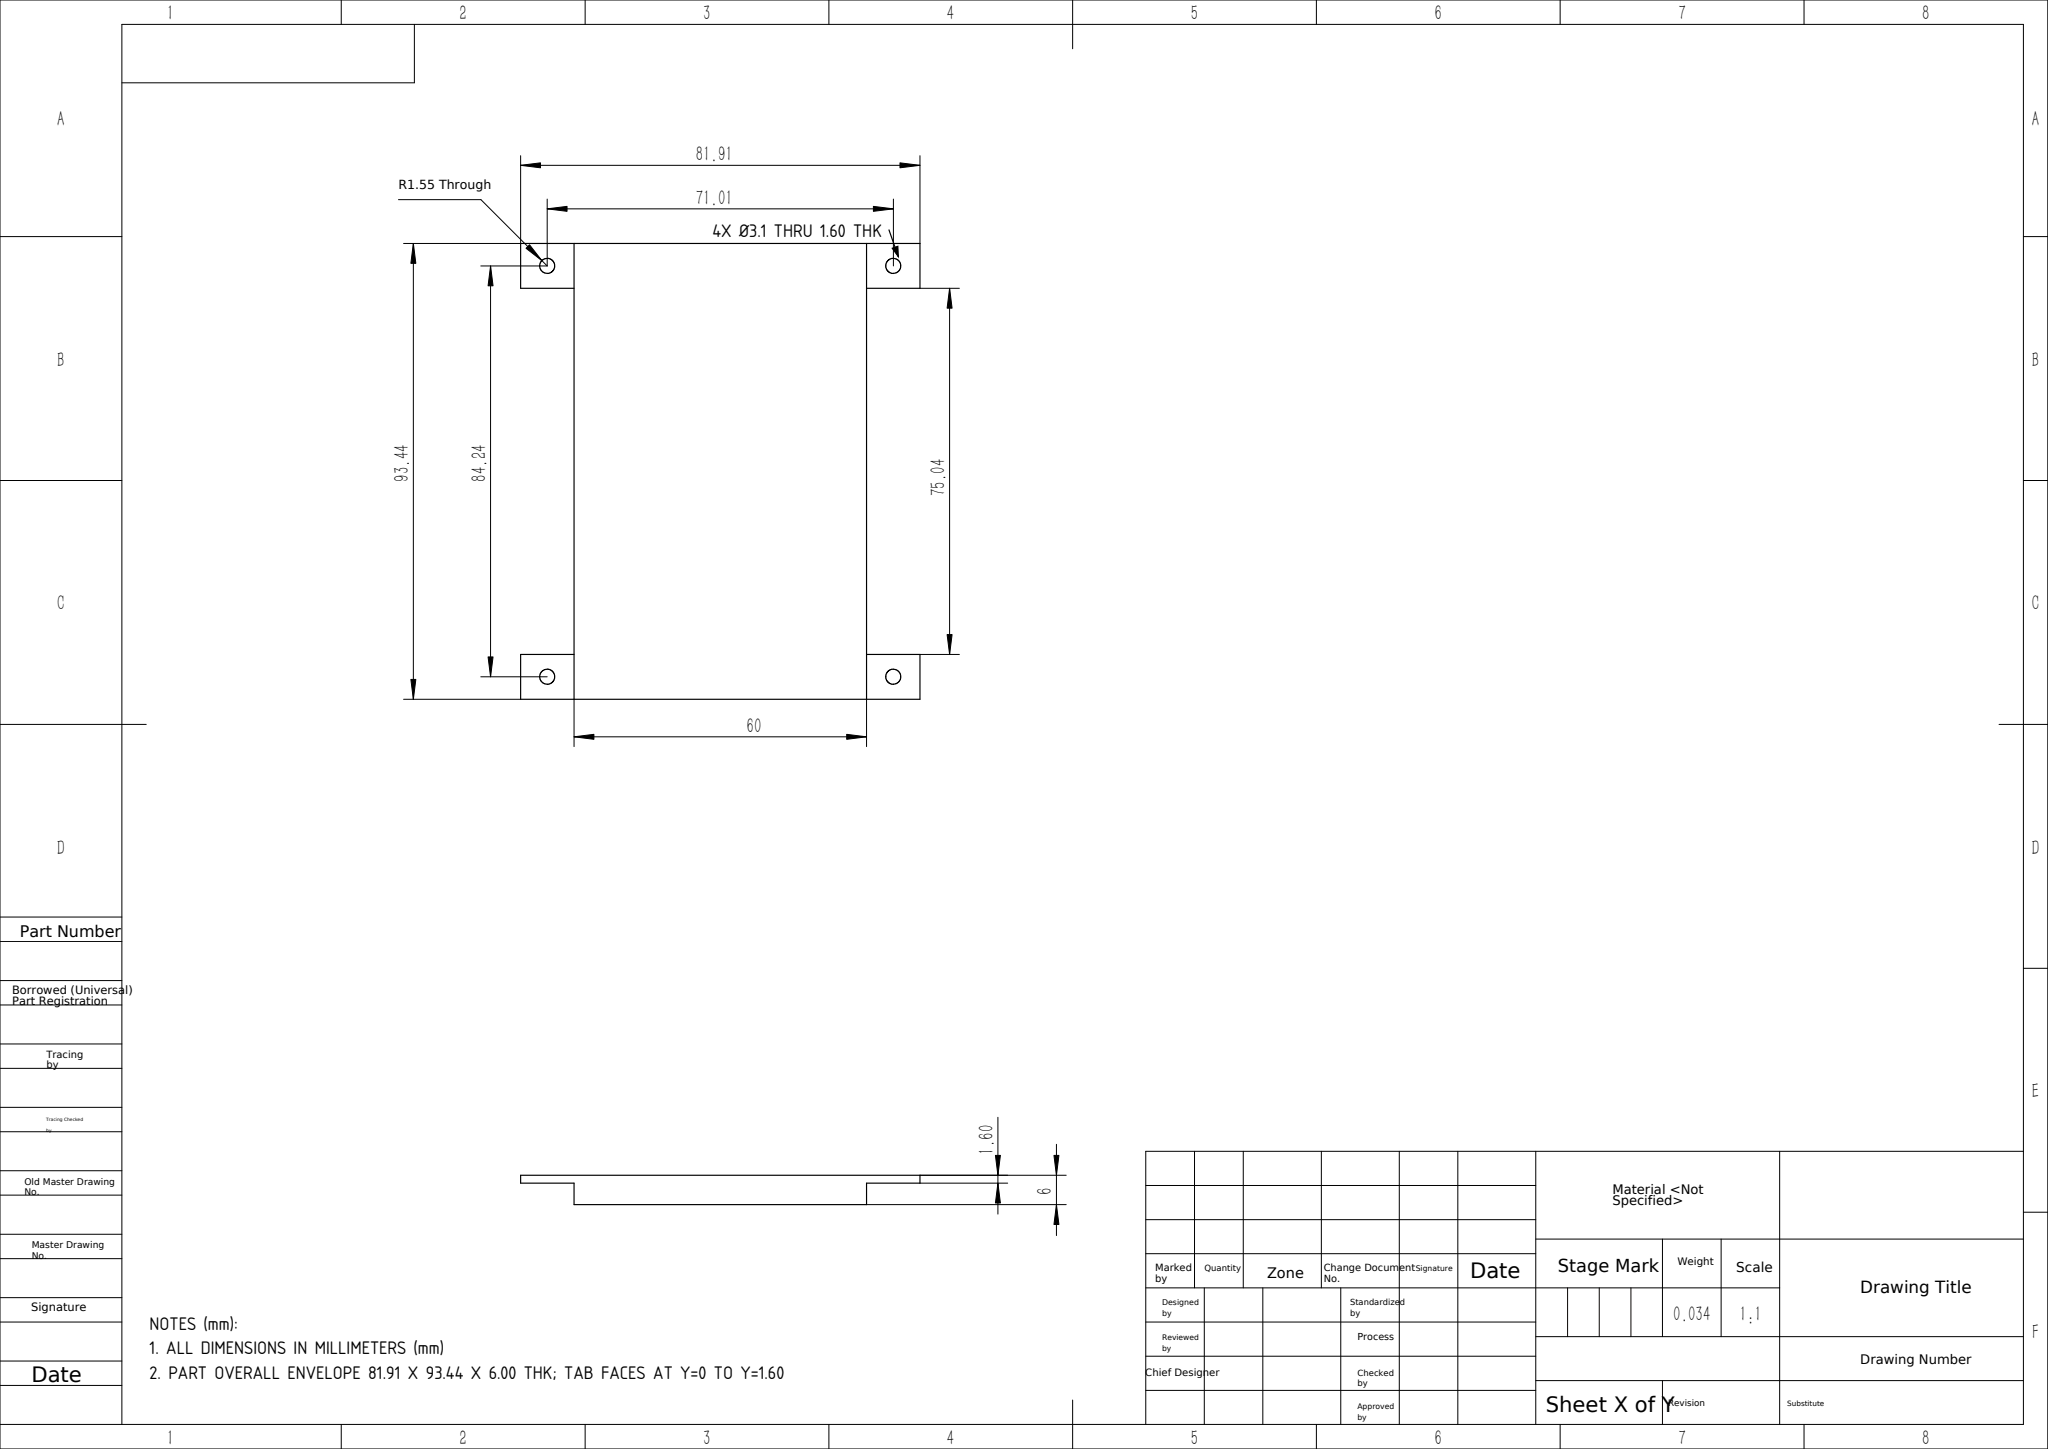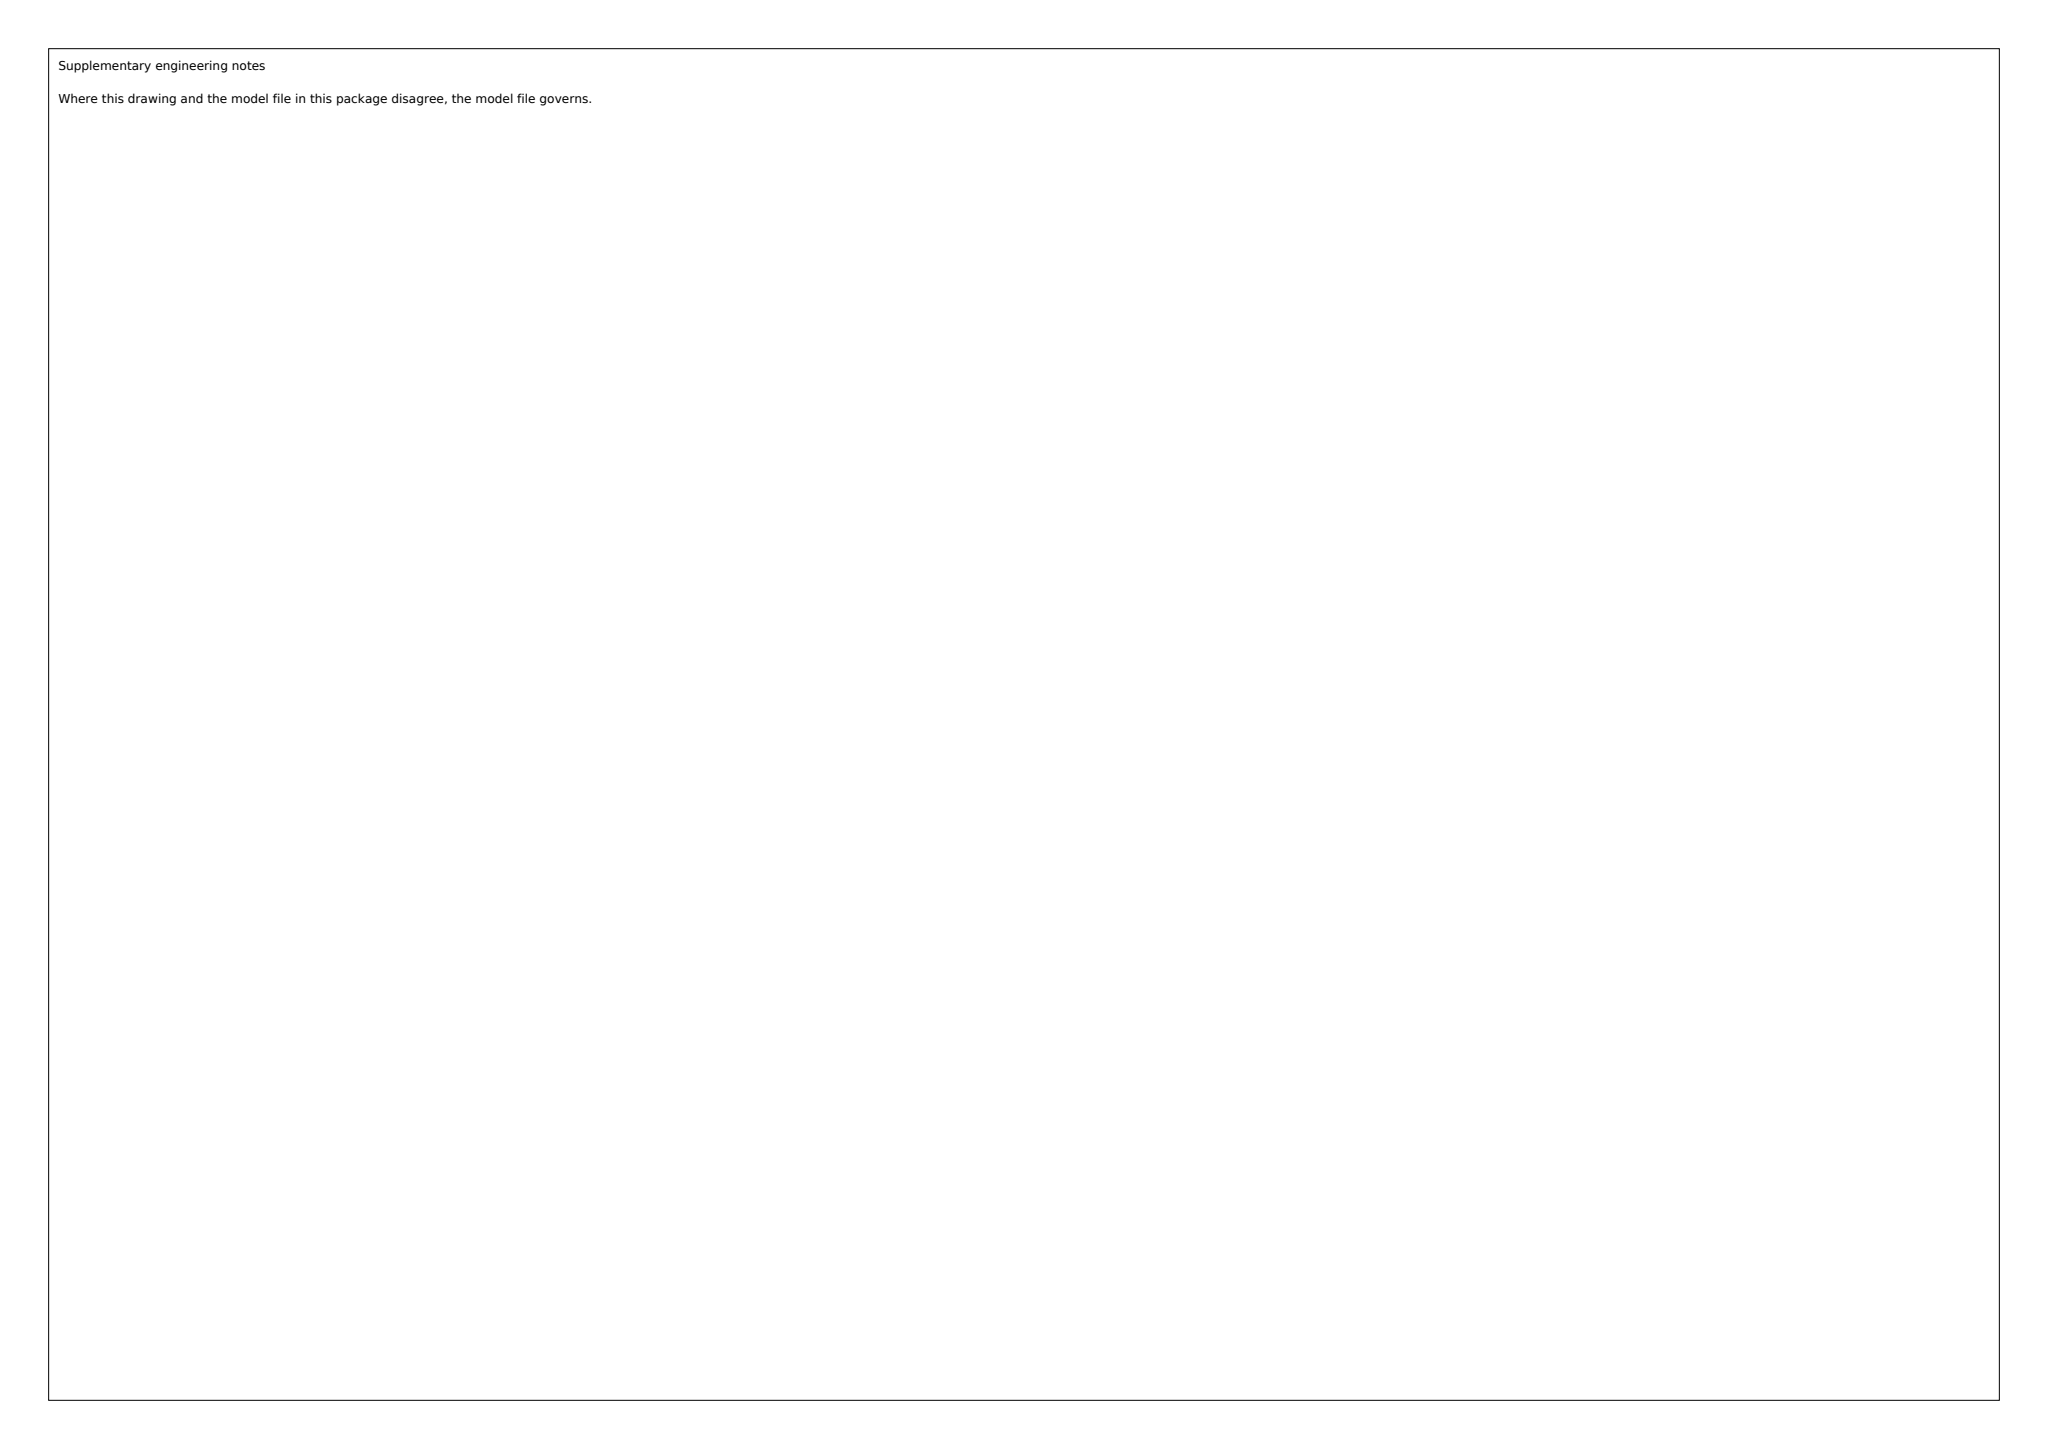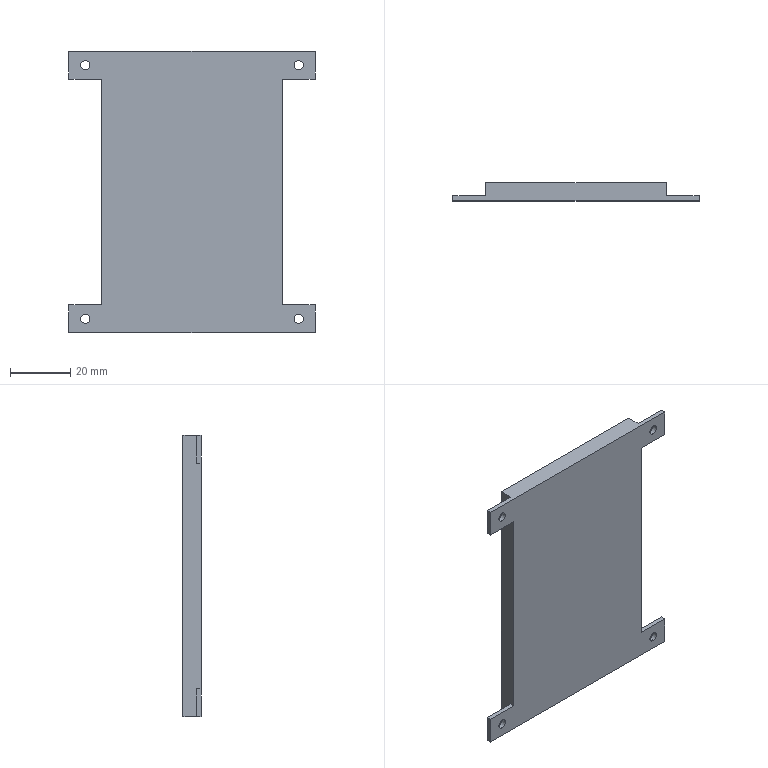Part | SolidWorks | mm | 1 solid | 26 faces | box 81.91 x 6 x 93.44 mm | volume 34235 mm3 | plane 18 | cylinder 8 | commonest cylinder face diameters 3.1 x8
Drawing notes:
ALL DIMENSIONS IN MILLIMETERS (mm) | from the solid: STEP bbox_xyz [81.91, 6.0, 93.44] given in mm
4X Ø3.1 THRU 1.60 THK MOUNTING TABS; HOLE CENTERS AT X=5.45 AND X=76.46 FROM LEFT EDGE, Z=4.60 AND Z=88.84 FROM BOTTOM EDGE | from the solid: cylinders dia 3.1, axis y, length 1.6 at (5.45,4.6), (5.45,88.84), (76.46,4.6), (76.46,88.84)
PART OVERALL ENVELOPE 81.91 X 93.44 X 6.00 THK; TAB FACES AT Y=0 TO Y=1.60 | from the solid: bbox_xyz [81.91, 6.0, 93.44]; y planes at 0.0, 1.6, 6.0
STEP:
#1=CARTESIAN_POINT('',(-35.505,0.,-43.67));
#2=VERTEX_POINT('',#1);
#3=CARTESIAN_POINT('',(-35.505,1.6,-43.67));
#4=VERTEX_POINT('',#3);
#5=CARTESIAN_POINT('',(-35.505,0.,-43.67));
#6=DIRECTION('',(0.,1.,0.));
#7=VECTOR('',#6,1000.);
#8=LINE('',#5,#7);
#9=EDGE_CURVE('',#2,#4,#8,.T.);
#10=ORIENTED_EDGE('',*,*,#9,.F.);
#11=CARTESIAN_POINT('',(-35.505,0.,-40.57));
#12=VERTEX_POINT('',#11);
#13=CARTESIAN_POINT('',(-35.505,0.,-42.12));
#14=DIRECTION('',(0.,-1.,0.));
#15=DIRECTION('',(0.,0.,1.));
#16=AXIS2_PLACEMENT_3D('',#13,#14,#15);
#17=CIRCLE('',#16,1.55);
#18=EDGE_CURVE('',#2,#12,#17,.T.);
#19=ORIENTED_EDGE('',*,*,#18,.T.);
#20=CARTESIAN_POINT('',(-35.505,1.6,-40.57));
#21=VERTEX_POINT('',#20);
#22=CARTESIAN_POINT('',(-35.505,0.,-40.57));
#23=DIRECTION('',(0.,1.,0.));
#24=VECTOR('',#23,1000.);
#25=LINE('',#22,#24);
#26=EDGE_CURVE('',#12,#21,#25,.T.);
#27=ORIENTED_EDGE('',*,*,#26,.T.);
#28=CARTESIAN_POINT('',(-35.505,1.6,-42.12));
#29=DIRECTION('',(0.,-1.,0.));
#30=DIRECTION('',(0.,0.,1.));
#31=AXIS2_PLACEMENT_3D('',#28,#29,#30);
#32=CIRCLE('',#31,1.55);
#33=EDGE_CURVE('',#4,#21,#32,.T.);
#34=ORIENTED_EDGE('',*,*,#33,.F.);
#35=EDGE_LOOP('',(#10,#19,#27,#34));
#36=FACE_OUTER_BOUND('',#35,.T.);
#37=CARTESIAN_POINT('',(-35.505,0.,-42.12));
#38=DIRECTION('',(0.,1.,0.));
#39=DIRECTION('',(0.,0.,1.));
#40=AXIS2_PLACEMENT_3D('',#37,#38,#39);
#41=CYLINDRICAL_SURFACE('',#40,1.55);
#42=ADVANCED_FACE('',(#36),#41,.F.);
#43=CARTESIAN_POINT('',(-35.505,0.,40.57));
#44=VERTEX_POINT('',#43);
#45=CARTESIAN_POINT('',(-35.505,1.6,40.57));
#46=VERTEX_POINT('',#45);
#47=CARTESIAN_POINT('',(-35.505,0.,40.57));
#48=DIRECTION('',(0.,1.,0.));
#49=VECTOR('',#48,1000.);
#50=LINE('',#47,#49);
#51=EDGE_CURVE('',#44,#46,#50,.T.);
#52=ORIENTED_EDGE('',*,*,#51,.F.);
#53=CARTESIAN_POINT('',(-35.505,0.,43.67));
#54=VERTEX_POINT('',#53);
#55=CARTESIAN_POINT('',(-35.505,0.,42.12));
#56=DIRECTION('',(0.,1.,0.));
#57=DIRECTION('',(0.,0.,-1.));
#58=AXIS2_PLACEMENT_3D('',#55,#56,#57);
#59=CIRCLE('',#58,1.55);
#60=EDGE_CURVE('',#54,#44,#59,.T.);
#61=ORIENTED_EDGE('',*,*,#60,.F.);
#62=CARTESIAN_POINT('',(-35.505,1.6,43.67));
#63=VERTEX_POINT('',#62);
#64=CARTESIAN_POINT('',(-35.505,0.,43.67));
#65=DIRECTION('',(0.,1.,0.));
#66=VECTOR('',#65,1000.);
#67=LINE('',#64,#66);
#68=EDGE_CURVE('',#54,#63,#67,.T.);
#69=ORIENTED_EDGE('',*,*,#68,.T.);
#70=CARTESIAN_POINT('',(-35.505,1.6,42.12));
#71=DIRECTION('',(0.,1.,0.));
#72=DIRECTION('',(0.,0.,-1.));
#73=AXIS2_PLACEMENT_3D('',#70,#71,#72);
#74=CIRCLE('',#73,1.55);
#75=EDGE_CURVE('',#63,#46,#74,.T.);
#76=ORIENTED_EDGE('',*,*,#75,.T.);
#77=EDGE_LOOP('',(#52,#61,#69,#76));
#78=FACE_OUTER_BOUND('',#77,.T.);
#79=CARTESIAN_POINT('',(-35.505,0.,42.12));
#80=DIRECTION('',(0.,1.,0.));
#81=DIRECTION('',(0.,0.,1.));
#82=AXIS2_PLACEMENT_3D('',#79,#80,#81);
#83=CYLINDRICAL_SURFACE('',#82,1.55);
#84=ADVANCED_FACE('',(#78),#83,.F.);
#85=CARTESIAN_POINT('',(35.505,0.,40.57));
#86=VERTEX_POINT('',#85);
#87=CARTESIAN_POINT('',(35.505,1.6,40.57));
#88=VERTEX_POINT('',#87);
#89=CARTESIAN_POINT('',(35.505,0.,40.57));
#90=DIRECTION('',(0.,1.,0.));
#91=VECTOR('',#90,1000.);
#92=LINE('',#89,#91);
#93=EDGE_CURVE('',#86,#88,#92,.T.);
#94=ORIENTED_EDGE('',*,*,#93,.F.);
#95=CARTESIAN_POINT('',(35.505,0.,43.67));
#96=VERTEX_POINT('',#95);
#97=CARTESIAN_POINT('',(35.505,0.,42.12));
#98=DIRECTION('',(0.,-1.,0.));
#99=DIRECTION('',(0.,0.,-1.));
#100=AXIS2_PLACEMENT_3D('',#97,#98,#99);
#101=CIRCLE('',#100,1.55);
#102=EDGE_CURVE('',#86,#96,#101,.T.);
#103=ORIENTED_EDGE('',*,*,#102,.T.);
#104=CARTESIAN_POINT('',(35.505,1.6,43.67));
#105=VERTEX_POINT('',#104);
#106=CARTESIAN_POINT('',(35.505,0.,43.67));
#107=DIRECTION('',(0.,1.,0.));
#108=VECTOR('',#107,1000.);
#109=LINE('',#106,#108);
#110=EDGE_CURVE('',#96,#105,#109,.T.);
#111=ORIENTED_EDGE('',*,*,#110,.T.);
#112=CARTESIAN_POINT('',(35.505,1.6,42.12));
#113=DIRECTION('',(0.,-1.,0.));
#114=DIRECTION('',(0.,0.,-1.));
#115=AXIS2_PLACEMENT_3D('',#112,#113,#114);
#116=CIRCLE('',#115,1.55);
#117=EDGE_CURVE('',#88,#105,#116,.T.);
#118=ORIENTED_EDGE('',*,*,#117,.F.);
#119=EDGE_LOOP('',(#94,#103,#111,#118));
#120=FACE_OUTER_BOUND('',#119,.T.);
#121=CARTESIAN_POINT('',(35.505,0.,42.12));
#122=DIRECTION('',(0.,1.,0.));
#123=DIRECTION('',(0.,0.,1.));
#124=AXIS2_PLACEMENT_3D('',#121,#122,#123);
#125=CYLINDRICAL_SURFACE('',#124,1.55);
#126=ADVANCED_FACE('',(#120),#125,.F.);
#127=CARTESIAN_POINT('',(35.505,0.,-43.67));
#128=VERTEX_POINT('',#127);
#129=CARTESIAN_POINT('',(35.505,1.6,-43.67));
#130=VERTEX_POINT('',#129);
#131=CARTESIAN_POINT('',(35.505,0.,-43.67));
#132=DIRECTION('',(0.,1.,0.));
#133=VECTOR('',#132,1000.);
#134=LINE('',#131,#133);
#135=EDGE_CURVE('',#128,#130,#134,.T.);
#136=ORIENTED_EDGE('',*,*,#135,.F.);
#137=CARTESIAN_POINT('',(35.505,0.,-40.57));
#138=VERTEX_POINT('',#137);
#139=CARTESIAN_POINT('',(35.505,0.,-42.12));
#140=DIRECTION('',(0.,1.,0.));
#141=DIRECTION('',(0.,0.,1.));
#142=AXIS2_PLACEMENT_3D('',#139,#140,#141);
#143=CIRCLE('',#142,1.55);
#144=EDGE_CURVE('',#138,#128,#143,.T.);
#145=ORIENTED_EDGE('',*,*,#144,.F.);
#146=CARTESIAN_POINT('',(35.505,1.6,-40.57));
#147=VERTEX_POINT('',#146);
#148=CARTESIAN_POINT('',(35.505,0.,-40.57));
#149=DIRECTION('',(0.,1.,0.));
#150=VECTOR('',#149,1000.);
#151=LINE('',#148,#150);
#152=EDGE_CURVE('',#138,#147,#151,.T.);
#153=ORIENTED_EDGE('',*,*,#152,.T.);
#154=CARTESIAN_POINT('',(35.505,1.6,-42.12));
#155=DIRECTION('',(0.,1.,0.));
#156=DIRECTION('',(0.,0.,1.));
#157=AXIS2_PLACEMENT_3D('',#154,#155,#156);
#158=CIRCLE('',#157,1.55);
#159=EDGE_CURVE('',#147,#130,#158,.T.);
#160=ORIENTED_EDGE('',*,*,#159,.T.);
#161=EDGE_LOOP('',(#136,#145,#153,#160));
#162=FACE_OUTER_BOUND('',#161,.T.);
#163=CARTESIAN_POINT('',(35.505,0.,-42.12));
#164=DIRECTION('',(0.,1.,0.));
#165=DIRECTION('',(0.,0.,1.));
#166=AXIS2_PLACEMENT_3D('',#163,#164,#165);
#167=CYLINDRICAL_SURFACE('',#166,1.55);
#168=ADVANCED_FACE('',(#162),#167,.F.);
#169=ORIENTED_EDGE('',*,*,#75,.F.);
#170=CARTESIAN_POINT('',(-35.505,1.6,42.12));
#171=DIRECTION('',(0.,1.,0.));
#172=DIRECTION('',(0.,0.,-1.));
#173=AXIS2_PLACEMENT_3D('',#170,#171,#172);
#174=CIRCLE('',#173,1.55);
#175=EDGE_CURVE('',#46,#63,#174,.T.);
#176=ORIENTED_EDGE('',*,*,#175,.F.);
#177=EDGE_LOOP('',(#169,#176));
#178=FACE_BOUND('',#177,.T.);
#179=CARTESIAN_POINT('',(-40.955,1.6,37.52));
#180=VERTEX_POINT('',#179);
#181=CARTESIAN_POINT('',(-30.,1.6,37.52));
#182=VERTEX_POINT('',#181);
#183=CARTESIAN_POINT('',(0.,1.6,37.52));
#184=DIRECTION('',(1.,0.,0.));
#185=VECTOR('',#184,1000.);
#186=LINE('',#183,#185);
#187=EDGE_CURVE('',#180,#182,#186,.T.);
#188=ORIENTED_EDGE('',*,*,#187,.F.);
#189=CARTESIAN_POINT('',(-40.955,1.6,46.72));
#190=VERTEX_POINT('',#189);
#191=CARTESIAN_POINT('',(-40.955,1.6,0.));
#192=DIRECTION('',(0.,0.,-1.));
#193=VECTOR('',#192,1000.);
#194=LINE('',#191,#193);
#195=EDGE_CURVE('',#190,#180,#194,.T.);
#196=ORIENTED_EDGE('',*,*,#195,.F.);
#197=CARTESIAN_POINT('',(-30.,1.6,46.72));
#198=VERTEX_POINT('',#197);
#199=CARTESIAN_POINT('',(0.,1.6,46.72));
#200=DIRECTION('',(-1.,0.,0.));
#201=VECTOR('',#200,1000.);
#202=LINE('',#199,#201);
#203=EDGE_CURVE('',#198,#190,#202,.T.);
#204=ORIENTED_EDGE('',*,*,#203,.F.);
#205=CARTESIAN_POINT('',(-30.,1.6,0.));
#206=DIRECTION('',(0.,0.,1.));
#207=VECTOR('',#206,1000.);
#208=LINE('',#205,#207);
#209=EDGE_CURVE('',#182,#198,#208,.T.);
#210=ORIENTED_EDGE('',*,*,#209,.F.);
#211=EDGE_LOOP('',(#188,#196,#204,#210));
#212=FACE_OUTER_BOUND('',#211,.T.);
#213=CARTESIAN_POINT('',(0.,1.6,0.));
#214=DIRECTION('',(0.,-1.,0.));
#215=DIRECTION('',(0.,0.,-1.));
#216=AXIS2_PLACEMENT_3D('',#213,#214,#215);
#217=PLANE('',#216);
#218=ADVANCED_FACE('',(#178,#212),#217,.F.);
#219=CARTESIAN_POINT('',(-40.955,0.,46.72));
#220=VERTEX_POINT('',#219);
#221=CARTESIAN_POINT('',(-40.955,0.,37.52));
#222=VERTEX_POINT('',#221);
#223=CARTESIAN_POINT('',(-40.955,0.,0.));
#224=DIRECTION('',(0.,0.,-1.));
#225=VECTOR('',#224,1000.);
#226=LINE('',#223,#225);
#227=EDGE_CURVE('',#220,#222,#226,.T.);
#228=ORIENTED_EDGE('',*,*,#227,.F.);
#229=CARTESIAN_POINT('',(-40.955,1.6,46.72));
#230=DIRECTION('',(0.,-1.,0.));
#231=VECTOR('',#230,1000.);
#232=LINE('',#229,#231);
#233=EDGE_CURVE('',#190,#220,#232,.T.);
#234=ORIENTED_EDGE('',*,*,#233,.F.);
#235=ORIENTED_EDGE('',*,*,#195,.T.);
#236=CARTESIAN_POINT('',(-40.955,1.6,37.52));
#237=DIRECTION('',(0.,-1.,0.));
#238=VECTOR('',#237,1000.);
#239=LINE('',#236,#238);
#240=EDGE_CURVE('',#180,#222,#239,.T.);
#241=ORIENTED_EDGE('',*,*,#240,.T.);
#242=EDGE_LOOP('',(#228,#234,#235,#241));
#243=FACE_OUTER_BOUND('',#242,.T.);
#244=CARTESIAN_POINT('',(-40.955,1.6,0.));
#245=DIRECTION('',(-1.,0.,0.));
#246=DIRECTION('',(0.,0.,1.));
#247=AXIS2_PLACEMENT_3D('',#244,#245,#246);
#248=PLANE('',#247);
#249=ADVANCED_FACE('',(#243),#248,.T.);
#250=CARTESIAN_POINT('',(-30.,0.,37.52));
#251=VERTEX_POINT('',#250);
#252=CARTESIAN_POINT('',(0.,0.,37.52));
#253=DIRECTION('',(1.,0.,0.));
#254=VECTOR('',#253,1000.);
#255=LINE('',#252,#254);
#256=EDGE_CURVE('',#222,#251,#255,.T.);
#257=ORIENTED_EDGE('',*,*,#256,.F.);
#258=ORIENTED_EDGE('',*,*,#240,.F.);
#259=ORIENTED_EDGE('',*,*,#187,.T.);
#260=CARTESIAN_POINT('',(-30.,1.6,37.52));
#261=DIRECTION('',(0.,-1.,0.));
#262=VECTOR('',#261,1000.);
#263=LINE('',#260,#262);
#264=EDGE_CURVE('',#182,#251,#263,.T.);
#265=ORIENTED_EDGE('',*,*,#264,.T.);
#266=EDGE_LOOP('',(#257,#258,#259,#265));
#267=FACE_OUTER_BOUND('',#266,.T.);
#268=CARTESIAN_POINT('',(0.,1.6,37.52));
#269=DIRECTION('',(0.,0.,-1.));
#270=DIRECTION('',(0.,-1.,0.));
#271=AXIS2_PLACEMENT_3D('',#268,#269,#270);
#272=PLANE('',#271);
#273=ADVANCED_FACE('',(#267),#272,.T.);
#274=CARTESIAN_POINT('',(-35.505,1.6,-42.12));
#275=DIRECTION('',(0.,-1.,0.));
#276=DIRECTION('',(0.,0.,1.));
#277=AXIS2_PLACEMENT_3D('',#274,#275,#276);
#278=CIRCLE('',#277,1.55);
#279=EDGE_CURVE('',#21,#4,#278,.T.);
#280=ORIENTED_EDGE('',*,*,#279,.T.);
#281=ORIENTED_EDGE('',*,*,#33,.T.);
#282=EDGE_LOOP('',(#280,#281));
#283=FACE_BOUND('',#282,.T.);
#284=CARTESIAN_POINT('',(-40.955,1.6,-37.52));
#285=VERTEX_POINT('',#284);
#286=CARTESIAN_POINT('',(-30.,1.6,-37.52));
#287=VERTEX_POINT('',#286);
#288=CARTESIAN_POINT('',(0.,1.6,-37.52));
#289=DIRECTION('',(1.,0.,0.));
#290=VECTOR('',#289,1000.);
#291=LINE('',#288,#290);
#292=EDGE_CURVE('',#285,#287,#291,.T.);
#293=ORIENTED_EDGE('',*,*,#292,.T.);
#294=CARTESIAN_POINT('',(-30.,1.6,-46.72));
#295=VERTEX_POINT('',#294);
#296=CARTESIAN_POINT('',(-30.,1.6,0.));
#297=DIRECTION('',(0.,0.,-1.));
#298=VECTOR('',#297,1000.);
#299=LINE('',#296,#298);
#300=EDGE_CURVE('',#287,#295,#299,.T.);
#301=ORIENTED_EDGE('',*,*,#300,.T.);
#302=CARTESIAN_POINT('',(-40.955,1.6,-46.72));
#303=VERTEX_POINT('',#302);
#304=CARTESIAN_POINT('',(0.,1.6,-46.72));
#305=DIRECTION('',(-1.,0.,0.));
#306=VECTOR('',#305,1000.);
#307=LINE('',#304,#306);
#308=EDGE_CURVE('',#295,#303,#307,.T.);
#309=ORIENTED_EDGE('',*,*,#308,.T.);
#310=CARTESIAN_POINT('',(-40.955,1.6,0.));
#311=DIRECTION('',(0.,0.,1.));
#312=VECTOR('',#311,1000.);
#313=LINE('',#310,#312);
#314=EDGE_CURVE('',#303,#285,#313,.T.);
#315=ORIENTED_EDGE('',*,*,#314,.T.);
#316=EDGE_LOOP('',(#293,#301,#309,#315));
#317=FACE_OUTER_BOUND('',#316,.T.);
#318=CARTESIAN_POINT('',(0.,1.6,0.));
#319=DIRECTION('',(0.,-1.,0.));
#320=DIRECTION('',(0.,0.,-1.));
#321=AXIS2_PLACEMENT_3D('',#318,#319,#320);
#322=PLANE('',#321);
#323=ADVANCED_FACE('',(#283,#317),#322,.F.);
#324=CARTESIAN_POINT('',(-40.955,0.,-46.72));
#325=VERTEX_POINT('',#324);
#326=CARTESIAN_POINT('',(-40.955,0.,-37.52));
#327=VERTEX_POINT('',#326);
#328=CARTESIAN_POINT('',(-40.955,0.,0.));
#329=DIRECTION('',(0.,0.,1.));
#330=VECTOR('',#329,1000.);
#331=LINE('',#328,#330);
#332=EDGE_CURVE('',#325,#327,#331,.T.);
#333=ORIENTED_EDGE('',*,*,#332,.T.);
#334=CARTESIAN_POINT('',(-40.955,1.6,-37.52));
#335=DIRECTION('',(0.,-1.,0.));
#336=VECTOR('',#335,1000.);
#337=LINE('',#334,#336);
#338=EDGE_CURVE('',#285,#327,#337,.T.);
#339=ORIENTED_EDGE('',*,*,#338,.F.);
#340=ORIENTED_EDGE('',*,*,#314,.F.);
#341=CARTESIAN_POINT('',(-40.955,1.6,-46.72));
#342=DIRECTION('',(0.,-1.,0.));
#343=VECTOR('',#342,1000.);
#344=LINE('',#341,#343);
#345=EDGE_CURVE('',#303,#325,#344,.T.);
#346=ORIENTED_EDGE('',*,*,#345,.T.);
#347=EDGE_LOOP('',(#333,#339,#340,#346));
#348=FACE_OUTER_BOUND('',#347,.T.);
#349=CARTESIAN_POINT('',(-40.955,1.6,0.));
#350=DIRECTION('',(1.,0.,0.));
#351=DIRECTION('',(0.,1.,0.));
#352=AXIS2_PLACEMENT_3D('',#349,#350,#351);
#353=PLANE('',#352);
#354=ADVANCED_FACE('',(#348),#353,.F.);
#355=CARTESIAN_POINT('',(-30.,0.,-37.52));
#356=VERTEX_POINT('',#355);
#357=CARTESIAN_POINT('',(0.,0.,-37.52));
#358=DIRECTION('',(1.,0.,0.));
#359=VECTOR('',#358,1000.);
#360=LINE('',#357,#359);
#361=EDGE_CURVE('',#327,#356,#360,.T.);
#362=ORIENTED_EDGE('',*,*,#361,.T.);
#363=CARTESIAN_POINT('',(-30.,1.6,-37.52));
#364=DIRECTION('',(0.,-1.,0.));
#365=VECTOR('',#364,1000.);
#366=LINE('',#363,#365);
#367=EDGE_CURVE('',#287,#356,#366,.T.);
#368=ORIENTED_EDGE('',*,*,#367,.F.);
#369=ORIENTED_EDGE('',*,*,#292,.F.);
#370=ORIENTED_EDGE('',*,*,#338,.T.);
#371=EDGE_LOOP('',(#362,#368,#369,#370));
#372=FACE_OUTER_BOUND('',#371,.T.);
#373=CARTESIAN_POINT('',(0.,1.6,-37.52));
#374=DIRECTION('',(0.,0.,-1.));
#375=DIRECTION('',(0.,-1.,0.));
#376=AXIS2_PLACEMENT_3D('',#373,#374,#375);
#377=PLANE('',#376);
#378=ADVANCED_FACE('',(#372),#377,.F.);
#379=ORIENTED_EDGE('',*,*,#159,.F.);
#380=CARTESIAN_POINT('',(35.505,1.6,-42.12));
#381=DIRECTION('',(0.,1.,0.));
#382=DIRECTION('',(0.,0.,1.));
#383=AXIS2_PLACEMENT_3D('',#380,#381,#382);
#384=CIRCLE('',#383,1.55);
#385=EDGE_CURVE('',#130,#147,#384,.T.);
#386=ORIENTED_EDGE('',*,*,#385,.F.);
#387=EDGE_LOOP('',(#379,#386));
#388=FACE_BOUND('',#387,.T.);
#389=CARTESIAN_POINT('',(40.955,1.6,-37.52));
#390=VERTEX_POINT('',#389);
#391=CARTESIAN_POINT('',(30.,1.6,-37.52));
#392=VERTEX_POINT('',#391);
#393=CARTESIAN_POINT('',(0.,1.6,-37.52));
#394=DIRECTION('',(-1.,0.,0.));
#395=VECTOR('',#394,1000.);
#396=LINE('',#393,#395);
#397=EDGE_CURVE('',#390,#392,#396,.T.);
#398=ORIENTED_EDGE('',*,*,#397,.F.);
#399=CARTESIAN_POINT('',(40.955,1.6,-46.72));
#400=VERTEX_POINT('',#399);
#401=CARTESIAN_POINT('',(40.955,1.6,0.));
#402=DIRECTION('',(0.,0.,1.));
#403=VECTOR('',#402,1000.);
#404=LINE('',#401,#403);
#405=EDGE_CURVE('',#400,#390,#404,.T.);
#406=ORIENTED_EDGE('',*,*,#405,.F.);
#407=CARTESIAN_POINT('',(30.,1.6,-46.72));
#408=VERTEX_POINT('',#407);
#409=CARTESIAN_POINT('',(0.,1.6,-46.72));
#410=DIRECTION('',(1.,0.,0.));
#411=VECTOR('',#410,1000.);
#412=LINE('',#409,#411);
#413=EDGE_CURVE('',#408,#400,#412,.T.);
#414=ORIENTED_EDGE('',*,*,#413,.F.);
#415=CARTESIAN_POINT('',(30.,1.6,0.));
#416=DIRECTION('',(0.,0.,-1.));
#417=VECTOR('',#416,1000.);
#418=LINE('',#415,#417);
#419=EDGE_CURVE('',#392,#408,#418,.T.);
#420=ORIENTED_EDGE('',*,*,#419,.F.);
#421=EDGE_LOOP('',(#398,#406,#414,#420));
#422=FACE_OUTER_BOUND('',#421,.T.);
#423=CARTESIAN_POINT('',(0.,1.6,0.));
#424=DIRECTION('',(0.,-1.,0.));
#425=DIRECTION('',(0.,0.,-1.));
#426=AXIS2_PLACEMENT_3D('',#423,#424,#425);
#427=PLANE('',#426);
#428=ADVANCED_FACE('',(#388,#422),#427,.F.);
#429=CARTESIAN_POINT('',(40.955,0.,-46.72));
#430=VERTEX_POINT('',#429);
#431=CARTESIAN_POINT('',(40.955,0.,-37.52));
#432=VERTEX_POINT('',#431);
#433=CARTESIAN_POINT('',(40.955,0.,0.));
#434=DIRECTION('',(0.,0.,1.));
#435=VECTOR('',#434,1000.);
#436=LINE('',#433,#435);
#437=EDGE_CURVE('',#430,#432,#436,.T.);
#438=ORIENTED_EDGE('',*,*,#437,.F.);
#439=CARTESIAN_POINT('',(40.955,1.6,-46.72));
#440=DIRECTION('',(0.,-1.,0.));
#441=VECTOR('',#440,1000.);
#442=LINE('',#439,#441);
#443=EDGE_CURVE('',#400,#430,#442,.T.);
#444=ORIENTED_EDGE('',*,*,#443,.F.);
#445=ORIENTED_EDGE('',*,*,#405,.T.);
#446=CARTESIAN_POINT('',(40.955,1.6,-37.52));
#447=DIRECTION('',(0.,-1.,0.));
#448=VECTOR('',#447,1000.);
#449=LINE('',#446,#448);
#450=EDGE_CURVE('',#390,#432,#449,.T.);
#451=ORIENTED_EDGE('',*,*,#450,.T.);
#452=EDGE_LOOP('',(#438,#444,#445,#451));
#453=FACE_OUTER_BOUND('',#452,.T.);
#454=CARTESIAN_POINT('',(40.955,1.6,0.));
#455=DIRECTION('',(1.,0.,0.));
#456=DIRECTION('',(0.,1.,0.));
#457=AXIS2_PLACEMENT_3D('',#454,#455,#456);
#458=PLANE('',#457);
#459=ADVANCED_FACE('',(#453),#458,.T.);
#460=CARTESIAN_POINT('',(30.,0.,-37.52));
#461=VERTEX_POINT('',#460);
#462=CARTESIAN_POINT('',(0.,0.,-37.52));
#463=DIRECTION('',(-1.,0.,0.));
#464=VECTOR('',#463,1000.);
#465=LINE('',#462,#464);
#466=EDGE_CURVE('',#432,#461,#465,.T.);
#467=ORIENTED_EDGE('',*,*,#466,.F.);
#468=ORIENTED_EDGE('',*,*,#450,.F.);
#469=ORIENTED_EDGE('',*,*,#397,.T.);
#470=CARTESIAN_POINT('',(30.,1.6,-37.52));
#471=DIRECTION('',(0.,-1.,0.));
#472=VECTOR('',#471,1000.);
#473=LINE('',#470,#472);
#474=EDGE_CURVE('',#392,#461,#473,.T.);
#475=ORIENTED_EDGE('',*,*,#474,.T.);
#476=EDGE_LOOP('',(#467,#468,#469,#475));
#477=FACE_OUTER_BOUND('',#476,.T.);
#478=CARTESIAN_POINT('',(0.,1.6,-37.52));
#479=DIRECTION('',(0.,0.,1.));
#480=DIRECTION('',(1.,0.,0.));
#481=AXIS2_PLACEMENT_3D('',#478,#479,#480);
#482=PLANE('',#481);
#483=ADVANCED_FACE('',(#477),#482,.T.);
#484=CARTESIAN_POINT('',(35.505,1.6,42.12));
#485=DIRECTION('',(0.,-1.,0.));
#486=DIRECTION('',(0.,0.,-1.));
#487=AXIS2_PLACEMENT_3D('',#484,#485,#486);
#488=CIRCLE('',#487,1.55);
#489=EDGE_CURVE('',#105,#88,#488,.T.);
#490=ORIENTED_EDGE('',*,*,#489,.T.);
#491=ORIENTED_EDGE('',*,*,#117,.T.);
#492=EDGE_LOOP('',(#490,#491));
#493=FACE_BOUND('',#492,.T.);
#494=CARTESIAN_POINT('',(40.955,1.6,37.52));
#495=VERTEX_POINT('',#494);
#496=CARTESIAN_POINT('',(30.,1.6,37.52));
#497=VERTEX_POINT('',#496);
#498=CARTESIAN_POINT('',(0.,1.6,37.52));
#499=DIRECTION('',(-1.,0.,0.));
#500=VECTOR('',#499,1000.);
#501=LINE('',#498,#500);
#502=EDGE_CURVE('',#495,#497,#501,.T.);
#503=ORIENTED_EDGE('',*,*,#502,.T.);
#504=CARTESIAN_POINT('',(30.,1.6,46.72));
#505=VERTEX_POINT('',#504);
#506=CARTESIAN_POINT('',(30.,1.6,0.));
#507=DIRECTION('',(0.,0.,1.));
#508=VECTOR('',#507,1000.);
#509=LINE('',#506,#508);
#510=EDGE_CURVE('',#497,#505,#509,.T.);
#511=ORIENTED_EDGE('',*,*,#510,.T.);
#512=CARTESIAN_POINT('',(40.955,1.6,46.72));
#513=VERTEX_POINT('',#512);
#514=CARTESIAN_POINT('',(0.,1.6,46.72));
#515=DIRECTION('',(1.,0.,0.));
#516=VECTOR('',#515,1000.);
#517=LINE('',#514,#516);
#518=EDGE_CURVE('',#505,#513,#517,.T.);
#519=ORIENTED_EDGE('',*,*,#518,.T.);
#520=CARTESIAN_POINT('',(40.955,1.6,0.));
#521=DIRECTION('',(0.,0.,-1.));
#522=VECTOR('',#521,1000.);
#523=LINE('',#520,#522);
#524=EDGE_CURVE('',#513,#495,#523,.T.);
#525=ORIENTED_EDGE('',*,*,#524,.T.);
#526=EDGE_LOOP('',(#503,#511,#519,#525));
#527=FACE_OUTER_BOUND('',#526,.T.);
#528=CARTESIAN_POINT('',(0.,1.6,0.));
#529=DIRECTION('',(0.,-1.,0.));
#530=DIRECTION('',(0.,0.,-1.));
#531=AXIS2_PLACEMENT_3D('',#528,#529,#530);
#532=PLANE('',#531);
#533=ADVANCED_FACE('',(#493,#527),#532,.F.);
#534=CARTESIAN_POINT('',(40.955,0.,46.72));
#535=VERTEX_POINT('',#534);
#536=CARTESIAN_POINT('',(40.955,0.,37.52));
#537=VERTEX_POINT('',#536);
#538=CARTESIAN_POINT('',(40.955,0.,0.));
#539=DIRECTION('',(0.,0.,-1.));
#540=VECTOR('',#539,1000.);
#541=LINE('',#538,#540);
#542=EDGE_CURVE('',#535,#537,#541,.T.);
#543=ORIENTED_EDGE('',*,*,#542,.T.);
#544=CARTESIAN_POINT('',(40.955,1.6,37.52));
#545=DIRECTION('',(0.,-1.,0.));
#546=VECTOR('',#545,1000.);
#547=LINE('',#544,#546);
#548=EDGE_CURVE('',#495,#537,#547,.T.);
#549=ORIENTED_EDGE('',*,*,#548,.F.);
#550=ORIENTED_EDGE('',*,*,#524,.F.);
#551=CARTESIAN_POINT('',(40.955,1.6,46.72));
#552=DIRECTION('',(0.,-1.,0.));
#553=VECTOR('',#552,1000.);
#554=LINE('',#551,#553);
#555=EDGE_CURVE('',#513,#535,#554,.T.);
#556=ORIENTED_EDGE('',*,*,#555,.T.);
#557=EDGE_LOOP('',(#543,#549,#550,#556));
#558=FACE_OUTER_BOUND('',#557,.T.);
#559=CARTESIAN_POINT('',(40.955,1.6,0.));
#560=DIRECTION('',(-1.,0.,0.));
#561=DIRECTION('',(0.,0.,1.));
#562=AXIS2_PLACEMENT_3D('',#559,#560,#561);
#563=PLANE('',#562);
#564=ADVANCED_FACE('',(#558),#563,.F.);
#565=CARTESIAN_POINT('',(30.,0.,37.52));
#566=VERTEX_POINT('',#565);
#567=CARTESIAN_POINT('',(0.,0.,37.52));
#568=DIRECTION('',(-1.,0.,0.));
#569=VECTOR('',#568,1000.);
#570=LINE('',#567,#569);
#571=EDGE_CURVE('',#537,#566,#570,.T.);
#572=ORIENTED_EDGE('',*,*,#571,.T.);
#573=CARTESIAN_POINT('',(30.,1.6,37.52));
#574=DIRECTION('',(0.,-1.,0.));
#575=VECTOR('',#574,1000.);
#576=LINE('',#573,#575);
#577=EDGE_CURVE('',#497,#566,#576,.T.);
#578=ORIENTED_EDGE('',*,*,#577,.F.);
#579=ORIENTED_EDGE('',*,*,#502,.F.);
#580=ORIENTED_EDGE('',*,*,#548,.T.);
#581=EDGE_LOOP('',(#572,#578,#579,#580));
#582=FACE_OUTER_BOUND('',#581,.T.);
#583=CARTESIAN_POINT('',(0.,1.6,37.52));
#584=DIRECTION('',(0.,0.,1.));
#585=DIRECTION('',(1.,0.,0.));
#586=AXIS2_PLACEMENT_3D('',#583,#584,#585);
#587=PLANE('',#586);
#588=ADVANCED_FACE('',(#582),#587,.F.);
#589=ORIENTED_EDGE('',*,*,#144,.T.);
#590=CARTESIAN_POINT('',(35.505,0.,-42.12));
#591=DIRECTION('',(0.,1.,0.));
#592=DIRECTION('',(0.,0.,1.));
#593=AXIS2_PLACEMENT_3D('',#590,#591,#592);
#594=CIRCLE('',#593,1.55);
#595=EDGE_CURVE('',#128,#138,#594,.T.);
#596=ORIENTED_EDGE('',*,*,#595,.T.);
#597=EDGE_LOOP('',(#589,#596));
#598=FACE_BOUND('',#597,.T.);
#599=CARTESIAN_POINT('',(35.505,0.,42.12));
#600=DIRECTION('',(0.,-1.,0.));
#601=DIRECTION('',(0.,0.,-1.));
#602=AXIS2_PLACEMENT_3D('',#599,#600,#601);
#603=CIRCLE('',#602,1.55);
#604=EDGE_CURVE('',#96,#86,#603,.T.);
#605=ORIENTED_EDGE('',*,*,#604,.F.);
#606=ORIENTED_EDGE('',*,*,#102,.F.);
#607=EDGE_LOOP('',(#605,#606));
#608=FACE_BOUND('',#607,.T.);
#609=ORIENTED_EDGE('',*,*,#60,.T.);
#610=CARTESIAN_POINT('',(-35.505,0.,42.12));
#611=DIRECTION('',(0.,1.,0.));
#612=DIRECTION('',(0.,0.,-1.));
#613=AXIS2_PLACEMENT_3D('',#610,#611,#612);
#614=CIRCLE('',#613,1.55);
#615=EDGE_CURVE('',#44,#54,#614,.T.);
#616=ORIENTED_EDGE('',*,*,#615,.T.);
#617=EDGE_LOOP('',(#609,#616));
#618=FACE_BOUND('',#617,.T.);
#619=CARTESIAN_POINT('',(-35.505,0.,-42.12));
#620=DIRECTION('',(0.,-1.,0.));
#621=DIRECTION('',(0.,0.,1.));
#622=AXIS2_PLACEMENT_3D('',#619,#620,#621);
#623=CIRCLE('',#622,1.55);
#624=EDGE_CURVE('',#12,#2,#623,.T.);
#625=ORIENTED_EDGE('',*,*,#624,.F.);
#626=ORIENTED_EDGE('',*,*,#18,.F.);
#627=EDGE_LOOP('',(#625,#626));
#628=FACE_BOUND('',#627,.T.);
#629=CARTESIAN_POINT('',(-30.,0.,-46.72));
#630=DIRECTION('',(0.,0.,1.));
#631=VECTOR('',#630,1000.);
#632=LINE('',#629,#631);
#633=EDGE_CURVE('',#356,#251,#632,.T.);
#634=ORIENTED_EDGE('',*,*,#633,.F.);
#635=ORIENTED_EDGE('',*,*,#361,.F.);
#636=ORIENTED_EDGE('',*,*,#332,.F.);
#637=CARTESIAN_POINT('',(30.,0.,-46.72));
#638=DIRECTION('',(-1.,0.,0.));
#639=VECTOR('',#638,1000.);
#640=LINE('',#637,#639);
#641=EDGE_CURVE('',#430,#325,#640,.T.);
#642=ORIENTED_EDGE('',*,*,#641,.F.);
#643=ORIENTED_EDGE('',*,*,#437,.T.);
#644=ORIENTED_EDGE('',*,*,#466,.T.);
#645=CARTESIAN_POINT('',(30.,0.,-46.72));
#646=DIRECTION('',(0.,0.,-1.));
#647=VECTOR('',#646,1000.);
#648=LINE('',#645,#647);
#649=EDGE_CURVE('',#566,#461,#648,.T.);
#650=ORIENTED_EDGE('',*,*,#649,.F.);
#651=ORIENTED_EDGE('',*,*,#571,.F.);
#652=ORIENTED_EDGE('',*,*,#542,.F.);
#653=CARTESIAN_POINT('',(30.,0.,46.72));
#654=DIRECTION('',(1.,0.,0.));
#655=VECTOR('',#654,1000.);
#656=LINE('',#653,#655);
#657=EDGE_CURVE('',#220,#535,#656,.T.);
#658=ORIENTED_EDGE('',*,*,#657,.F.);
#659=ORIENTED_EDGE('',*,*,#227,.T.);
#660=ORIENTED_EDGE('',*,*,#256,.T.);
#661=EDGE_LOOP('',(#634,#635,#636,#642,#643,#644,#650,#651,#652,#658,#659,#660));
#662=FACE_OUTER_BOUND('',#661,.T.);
#663=CARTESIAN_POINT('',(0.,0.,0.));
#664=DIRECTION('',(0.,-1.,0.));
#665=DIRECTION('',(0.,0.,-1.));
#666=AXIS2_PLACEMENT_3D('',#663,#664,#665);
#667=PLANE('',#666);
#668=ADVANCED_FACE('',(#598,#608,#618,#628,#662),#667,.T.);
#669=CARTESIAN_POINT('',(-30.,6.,-46.72));
#670=VERTEX_POINT('',#669);
#671=CARTESIAN_POINT('',(-30.,6.,46.72));
#672=VERTEX_POINT('',#671);
#673=CARTESIAN_POINT('',(-30.,6.,-46.72));
#674=DIRECTION('',(0.,0.,1.));
#675=VECTOR('',#674,1000.);
#676=LINE('',#673,#675);
#677=EDGE_CURVE('',#670,#672,#676,.T.);
#678=ORIENTED_EDGE('',*,*,#677,.T.);
#679=CARTESIAN_POINT('',(30.,6.,46.72));
#680=VERTEX_POINT('',#679);
#681=CARTESIAN_POINT('',(30.,6.,46.72));
#682=DIRECTION('',(1.,0.,0.));
#683=VECTOR('',#682,1000.);
#684=LINE('',#681,#683);
#685=EDGE_CURVE('',#672,#680,#684,.T.);
#686=ORIENTED_EDGE('',*,*,#685,.T.);
#687=CARTESIAN_POINT('',(30.,6.,-46.72));
#688=VERTEX_POINT('',#687);
#689=CARTESIAN_POINT('',(30.,6.,-46.72));
#690=DIRECTION('',(0.,0.,-1.));
#691=VECTOR('',#690,1000.);
#692=LINE('',#689,#691);
#693=EDGE_CURVE('',#680,#688,#692,.T.);
#694=ORIENTED_EDGE('',*,*,#693,.T.);
#695=CARTESIAN_POINT('',(30.,6.,-46.72));
#696=DIRECTION('',(-1.,0.,0.));
#697=VECTOR('',#696,1000.);
#698=LINE('',#695,#697);
#699=EDGE_CURVE('',#688,#670,#698,.T.);
#700=ORIENTED_EDGE('',*,*,#699,.T.);
#701=EDGE_LOOP('',(#678,#686,#694,#700));
#702=FACE_OUTER_BOUND('',#701,.T.);
#703=CARTESIAN_POINT('',(0.,6.,0.));
#704=DIRECTION('',(0.,-1.,0.));
#705=DIRECTION('',(0.,0.,-1.));
#706=AXIS2_PLACEMENT_3D('',#703,#704,#705);
#707=PLANE('',#706);
#708=ADVANCED_FACE('',(#702),#707,.F.);
#709=ORIENTED_EDGE('',*,*,#641,.T.);
#710=ORIENTED_EDGE('',*,*,#345,.F.);
#711=ORIENTED_EDGE('',*,*,#308,.F.);
#712=CARTESIAN_POINT('',(-30.,6.,-46.72));
#713=DIRECTION('',(0.,-1.,0.));
#714=VECTOR('',#713,1000.);
#715=LINE('',#712,#714);
#716=EDGE_CURVE('',#670,#295,#715,.T.);
#717=ORIENTED_EDGE('',*,*,#716,.F.);
#718=ORIENTED_EDGE('',*,*,#699,.F.);
#719=CARTESIAN_POINT('',(30.,6.,-46.72));
#720=DIRECTION('',(0.,-1.,0.));
#721=VECTOR('',#720,1000.);
#722=LINE('',#719,#721);
#723=EDGE_CURVE('',#688,#408,#722,.T.);
#724=ORIENTED_EDGE('',*,*,#723,.T.);
#725=ORIENTED_EDGE('',*,*,#413,.T.);
#726=ORIENTED_EDGE('',*,*,#443,.T.);
#727=EDGE_LOOP('',(#709,#710,#711,#717,#718,#724,#725,#726));
#728=FACE_OUTER_BOUND('',#727,.T.);
#729=CARTESIAN_POINT('',(30.,6.,-46.72));
#730=DIRECTION('',(0.,0.,1.));
#731=DIRECTION('',(1.,0.,0.));
#732=AXIS2_PLACEMENT_3D('',#729,#730,#731);
#733=PLANE('',#732);
#734=ADVANCED_FACE('',(#728),#733,.F.);
#735=ORIENTED_EDGE('',*,*,#657,.T.);
#736=ORIENTED_EDGE('',*,*,#555,.F.);
#737=ORIENTED_EDGE('',*,*,#518,.F.);
#738=CARTESIAN_POINT('',(30.,6.,46.72));
#739=DIRECTION('',(0.,-1.,0.));
#740=VECTOR('',#739,1000.);
#741=LINE('',#738,#740);
#742=EDGE_CURVE('',#680,#505,#741,.T.);
#743=ORIENTED_EDGE('',*,*,#742,.F.);
#744=ORIENTED_EDGE('',*,*,#685,.F.);
#745=CARTESIAN_POINT('',(-30.,6.,46.72));
#746=DIRECTION('',(0.,-1.,0.));
#747=VECTOR('',#746,1000.);
#748=LINE('',#745,#747);
#749=EDGE_CURVE('',#672,#198,#748,.T.);
#750=ORIENTED_EDGE('',*,*,#749,.T.);
#751=ORIENTED_EDGE('',*,*,#203,.T.);
#752=ORIENTED_EDGE('',*,*,#233,.T.);
#753=EDGE_LOOP('',(#735,#736,#737,#743,#744,#750,#751,#752));
#754=FACE_OUTER_BOUND('',#753,.T.);
#755=CARTESIAN_POINT('',(30.,6.,46.72));
#756=DIRECTION('',(0.,0.,-1.));
#757=DIRECTION('',(0.,-1.,0.));
#758=AXIS2_PLACEMENT_3D('',#755,#756,#757);
#759=PLANE('',#758);
#760=ADVANCED_FACE('',(#754),#759,.F.);
#761=ORIENTED_EDGE('',*,*,#649,.T.);
#762=ORIENTED_EDGE('',*,*,#474,.F.);
#763=ORIENTED_EDGE('',*,*,#419,.T.);
#764=ORIENTED_EDGE('',*,*,#723,.F.);
#765=ORIENTED_EDGE('',*,*,#693,.F.);
#766=ORIENTED_EDGE('',*,*,#742,.T.);
#767=ORIENTED_EDGE('',*,*,#510,.F.);
#768=ORIENTED_EDGE('',*,*,#577,.T.);
#769=EDGE_LOOP('',(#761,#762,#763,#764,#765,#766,#767,#768));
#770=FACE_OUTER_BOUND('',#769,.T.);
#771=CARTESIAN_POINT('',(30.,6.,-46.72));
#772=DIRECTION('',(-1.,0.,0.));
#773=DIRECTION('',(0.,0.,1.));
#774=AXIS2_PLACEMENT_3D('',#771,#772,#773);
#775=PLANE('',#774);
#776=ADVANCED_FACE('',(#770),#775,.F.);
#777=ORIENTED_EDGE('',*,*,#633,.T.);
#778=ORIENTED_EDGE('',*,*,#264,.F.);
#779=ORIENTED_EDGE('',*,*,#209,.T.);
#780=ORIENTED_EDGE('',*,*,#749,.F.);
#781=ORIENTED_EDGE('',*,*,#677,.F.);
#782=ORIENTED_EDGE('',*,*,#716,.T.);
#783=ORIENTED_EDGE('',*,*,#300,.F.);
#784=ORIENTED_EDGE('',*,*,#367,.T.);
#785=EDGE_LOOP('',(#777,#778,#779,#780,#781,#782,#783,#784));
#786=FACE_OUTER_BOUND('',#785,.T.);
#787=CARTESIAN_POINT('',(-30.,6.,-46.72));
#788=DIRECTION('',(1.,0.,0.));
#789=DIRECTION('',(0.,1.,0.));
#790=AXIS2_PLACEMENT_3D('',#787,#788,#789);
#791=PLANE('',#790);
#792=ADVANCED_FACE('',(#786),#791,.F.);
#793=ORIENTED_EDGE('',*,*,#595,.F.);
#794=ORIENTED_EDGE('',*,*,#135,.T.);
#795=ORIENTED_EDGE('',*,*,#385,.T.);
#796=ORIENTED_EDGE('',*,*,#152,.F.);
#797=EDGE_LOOP('',(#793,#794,#795,#796));
#798=FACE_OUTER_BOUND('',#797,.T.);
#799=CARTESIAN_POINT('',(35.505,0.,-42.12));
#800=DIRECTION('',(0.,1.,0.));
#801=DIRECTION('',(0.,0.,1.));
#802=AXIS2_PLACEMENT_3D('',#799,#800,#801);
#803=CYLINDRICAL_SURFACE('',#802,1.55);
#804=ADVANCED_FACE('',(#798),#803,.F.);
#805=ORIENTED_EDGE('',*,*,#604,.T.);
#806=ORIENTED_EDGE('',*,*,#93,.T.);
#807=ORIENTED_EDGE('',*,*,#489,.F.);
#808=ORIENTED_EDGE('',*,*,#110,.F.);
#809=EDGE_LOOP('',(#805,#806,#807,#808));
#810=FACE_OUTER_BOUND('',#809,.T.);
#811=CARTESIAN_POINT('',(35.505,0.,42.12));
#812=DIRECTION('',(0.,1.,0.));
#813=DIRECTION('',(0.,0.,1.));
#814=AXIS2_PLACEMENT_3D('',#811,#812,#813);
#815=CYLINDRICAL_SURFACE('',#814,1.55);
#816=ADVANCED_FACE('',(#810),#815,.F.);
#817=ORIENTED_EDGE('',*,*,#615,.F.);
#818=ORIENTED_EDGE('',*,*,#51,.T.);
#819=ORIENTED_EDGE('',*,*,#175,.T.);
#820=ORIENTED_EDGE('',*,*,#68,.F.);
#821=EDGE_LOOP('',(#817,#818,#819,#820));
#822=FACE_OUTER_BOUND('',#821,.T.);
#823=CARTESIAN_POINT('',(-35.505,0.,42.12));
#824=DIRECTION('',(0.,1.,0.));
#825=DIRECTION('',(0.,0.,1.));
#826=AXIS2_PLACEMENT_3D('',#823,#824,#825);
#827=CYLINDRICAL_SURFACE('',#826,1.55);
#828=ADVANCED_FACE('',(#822),#827,.F.);
#829=ORIENTED_EDGE('',*,*,#624,.T.);
#830=ORIENTED_EDGE('',*,*,#9,.T.);
#831=ORIENTED_EDGE('',*,*,#279,.F.);
#832=ORIENTED_EDGE('',*,*,#26,.F.);
#833=EDGE_LOOP('',(#829,#830,#831,#832));
#834=FACE_OUTER_BOUND('',#833,.T.);
#835=CARTESIAN_POINT('',(-35.505,0.,-42.12));
#836=DIRECTION('',(0.,1.,0.));
#837=DIRECTION('',(0.,0.,1.));
#838=AXIS2_PLACEMENT_3D('',#835,#836,#837);
#839=CYLINDRICAL_SURFACE('',#838,1.55);
#840=ADVANCED_FACE('',(#834),#839,.F.);
#841=CLOSED_SHELL('',(#42,#84,#126,#168,#218,#249,#273,#323,#354,#378,#428,#459,#483,#533,#564,#588,#668,#708,#734,#760,#776,#792,#804,#816,#828,#840));
#842=MANIFOLD_SOLID_BREP('',#841);
#843=CARTESIAN_POINT('',(0.,0.,0.));
#844=DIRECTION('',(0.,0.,1.));
#845=DIRECTION('',(1.,0.,0.));
#846=AXIS2_PLACEMENT_3D('',#843,#844,#845);
#847=(LENGTH_UNIT()NAMED_UNIT(*)SI_UNIT(.MILLI.,.METRE.));
#848=UNCERTAINTY_MEASURE_WITH_UNIT(LENGTH_MEASURE(0.00001),#847,'','');
#849=(NAMED_UNIT(*)PLANE_ANGLE_UNIT()SI_UNIT($,.RADIAN.));
#850=(NAMED_UNIT(*)SI_UNIT($,.STERADIAN.)SOLID_ANGLE_UNIT());
#851=(GEOMETRIC_REPRESENTATION_CONTEXT(3)GLOBAL_UNCERTAINTY_ASSIGNED_CONTEXT((#848))GLOBAL_UNIT_ASSIGNED_CONTEXT((#847,#849,#850))REPRESENTATION_CONTEXT('',''));
#852=ADVANCED_BREP_SHAPE_REPRESENTATION('',(#842,#846),#851);